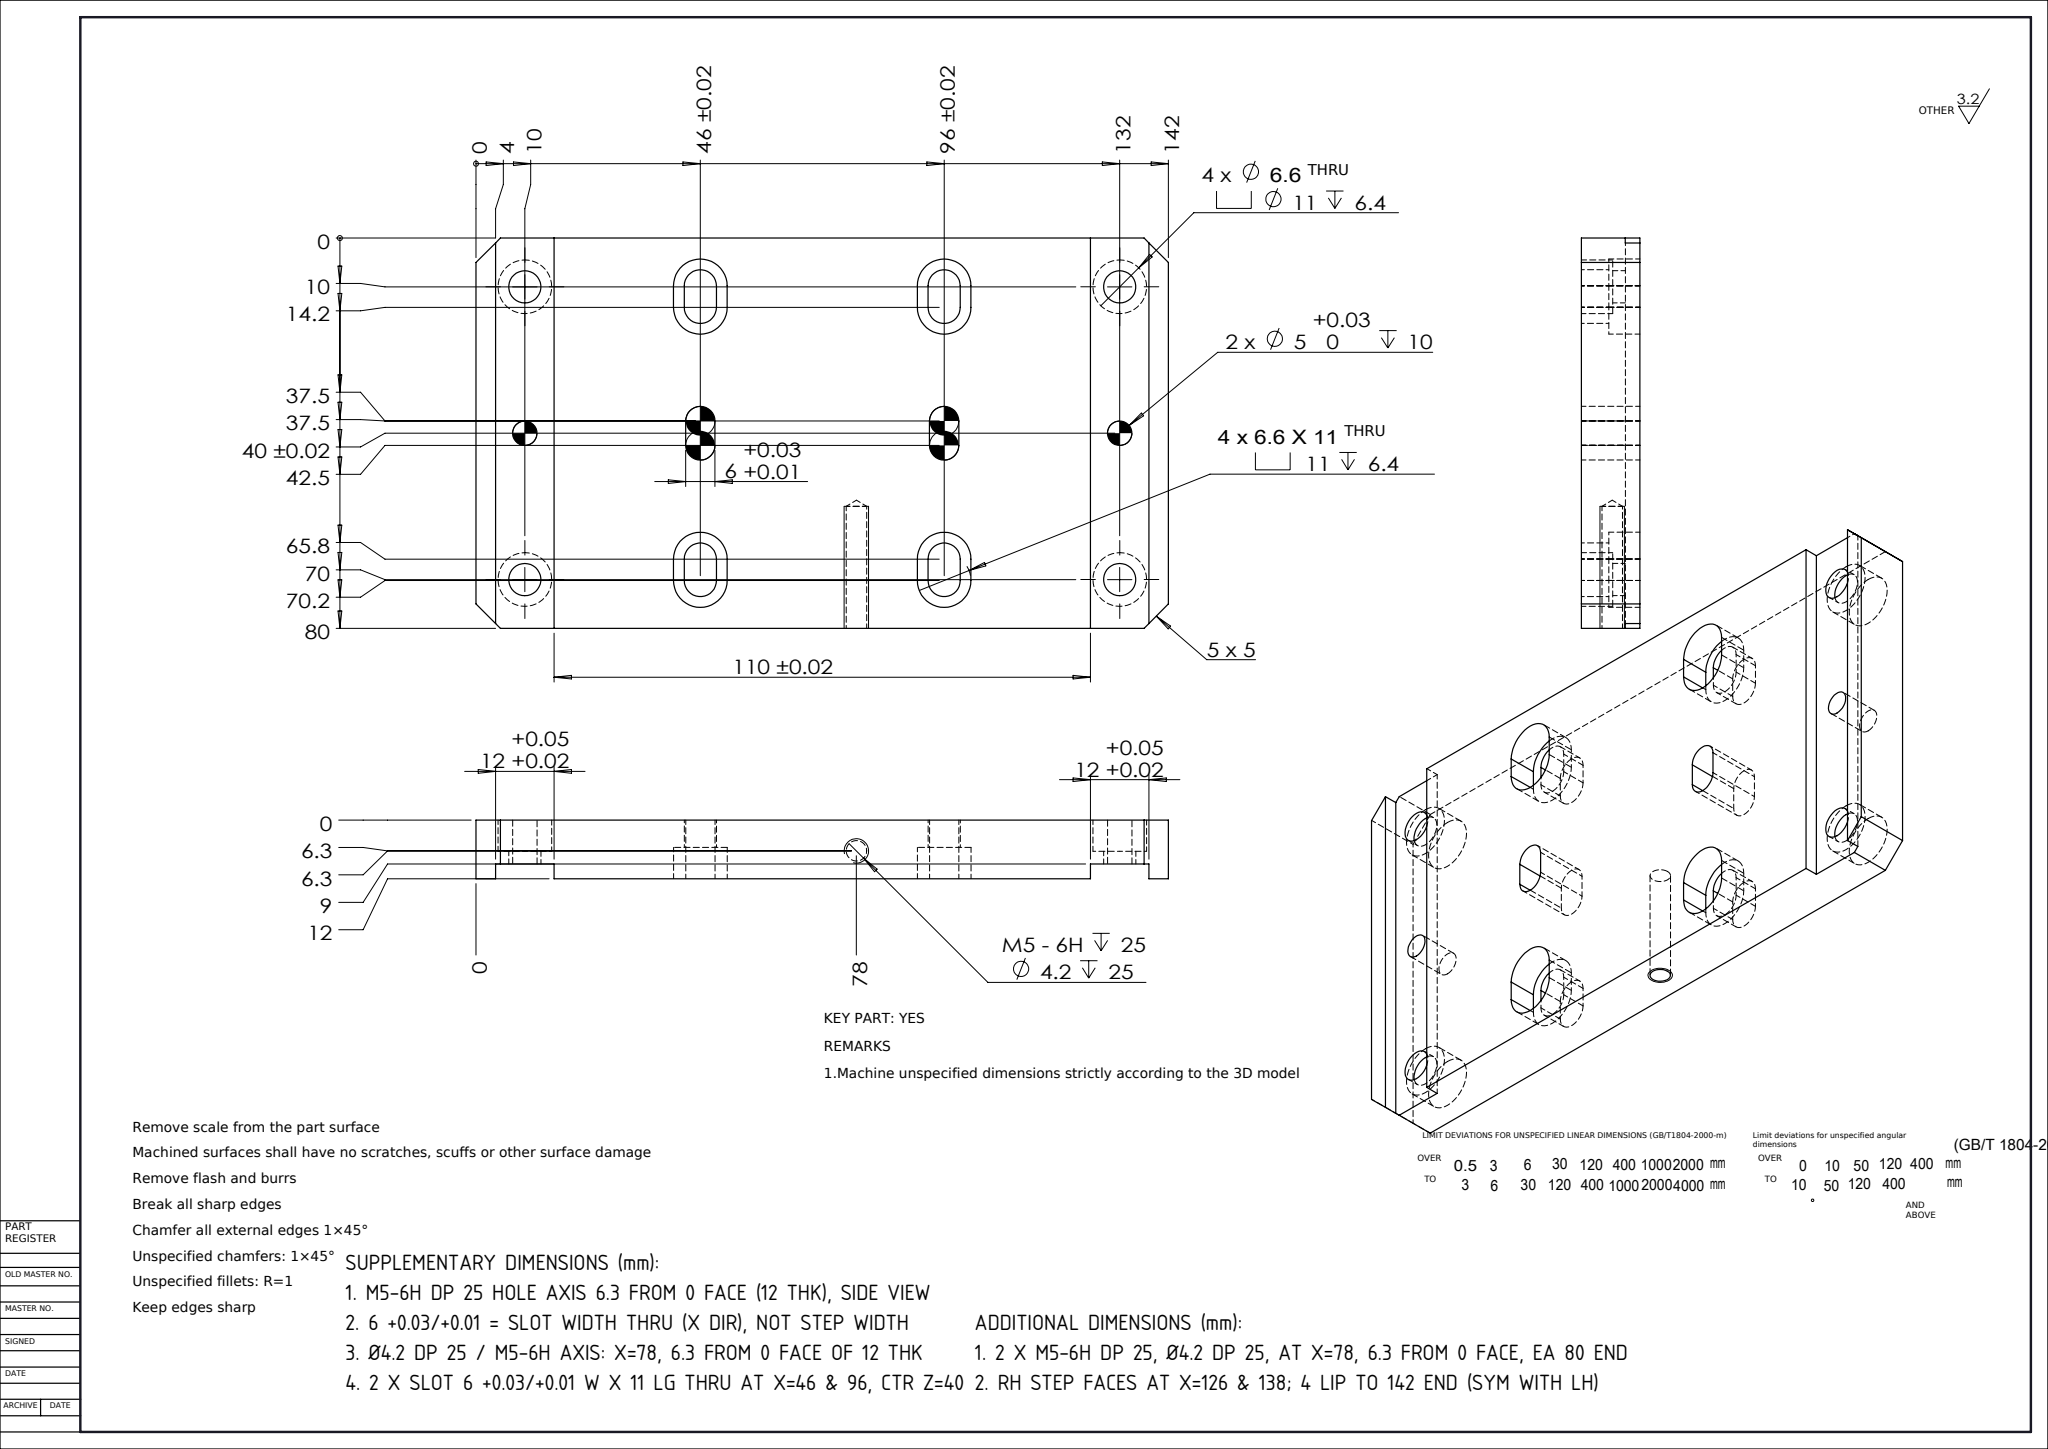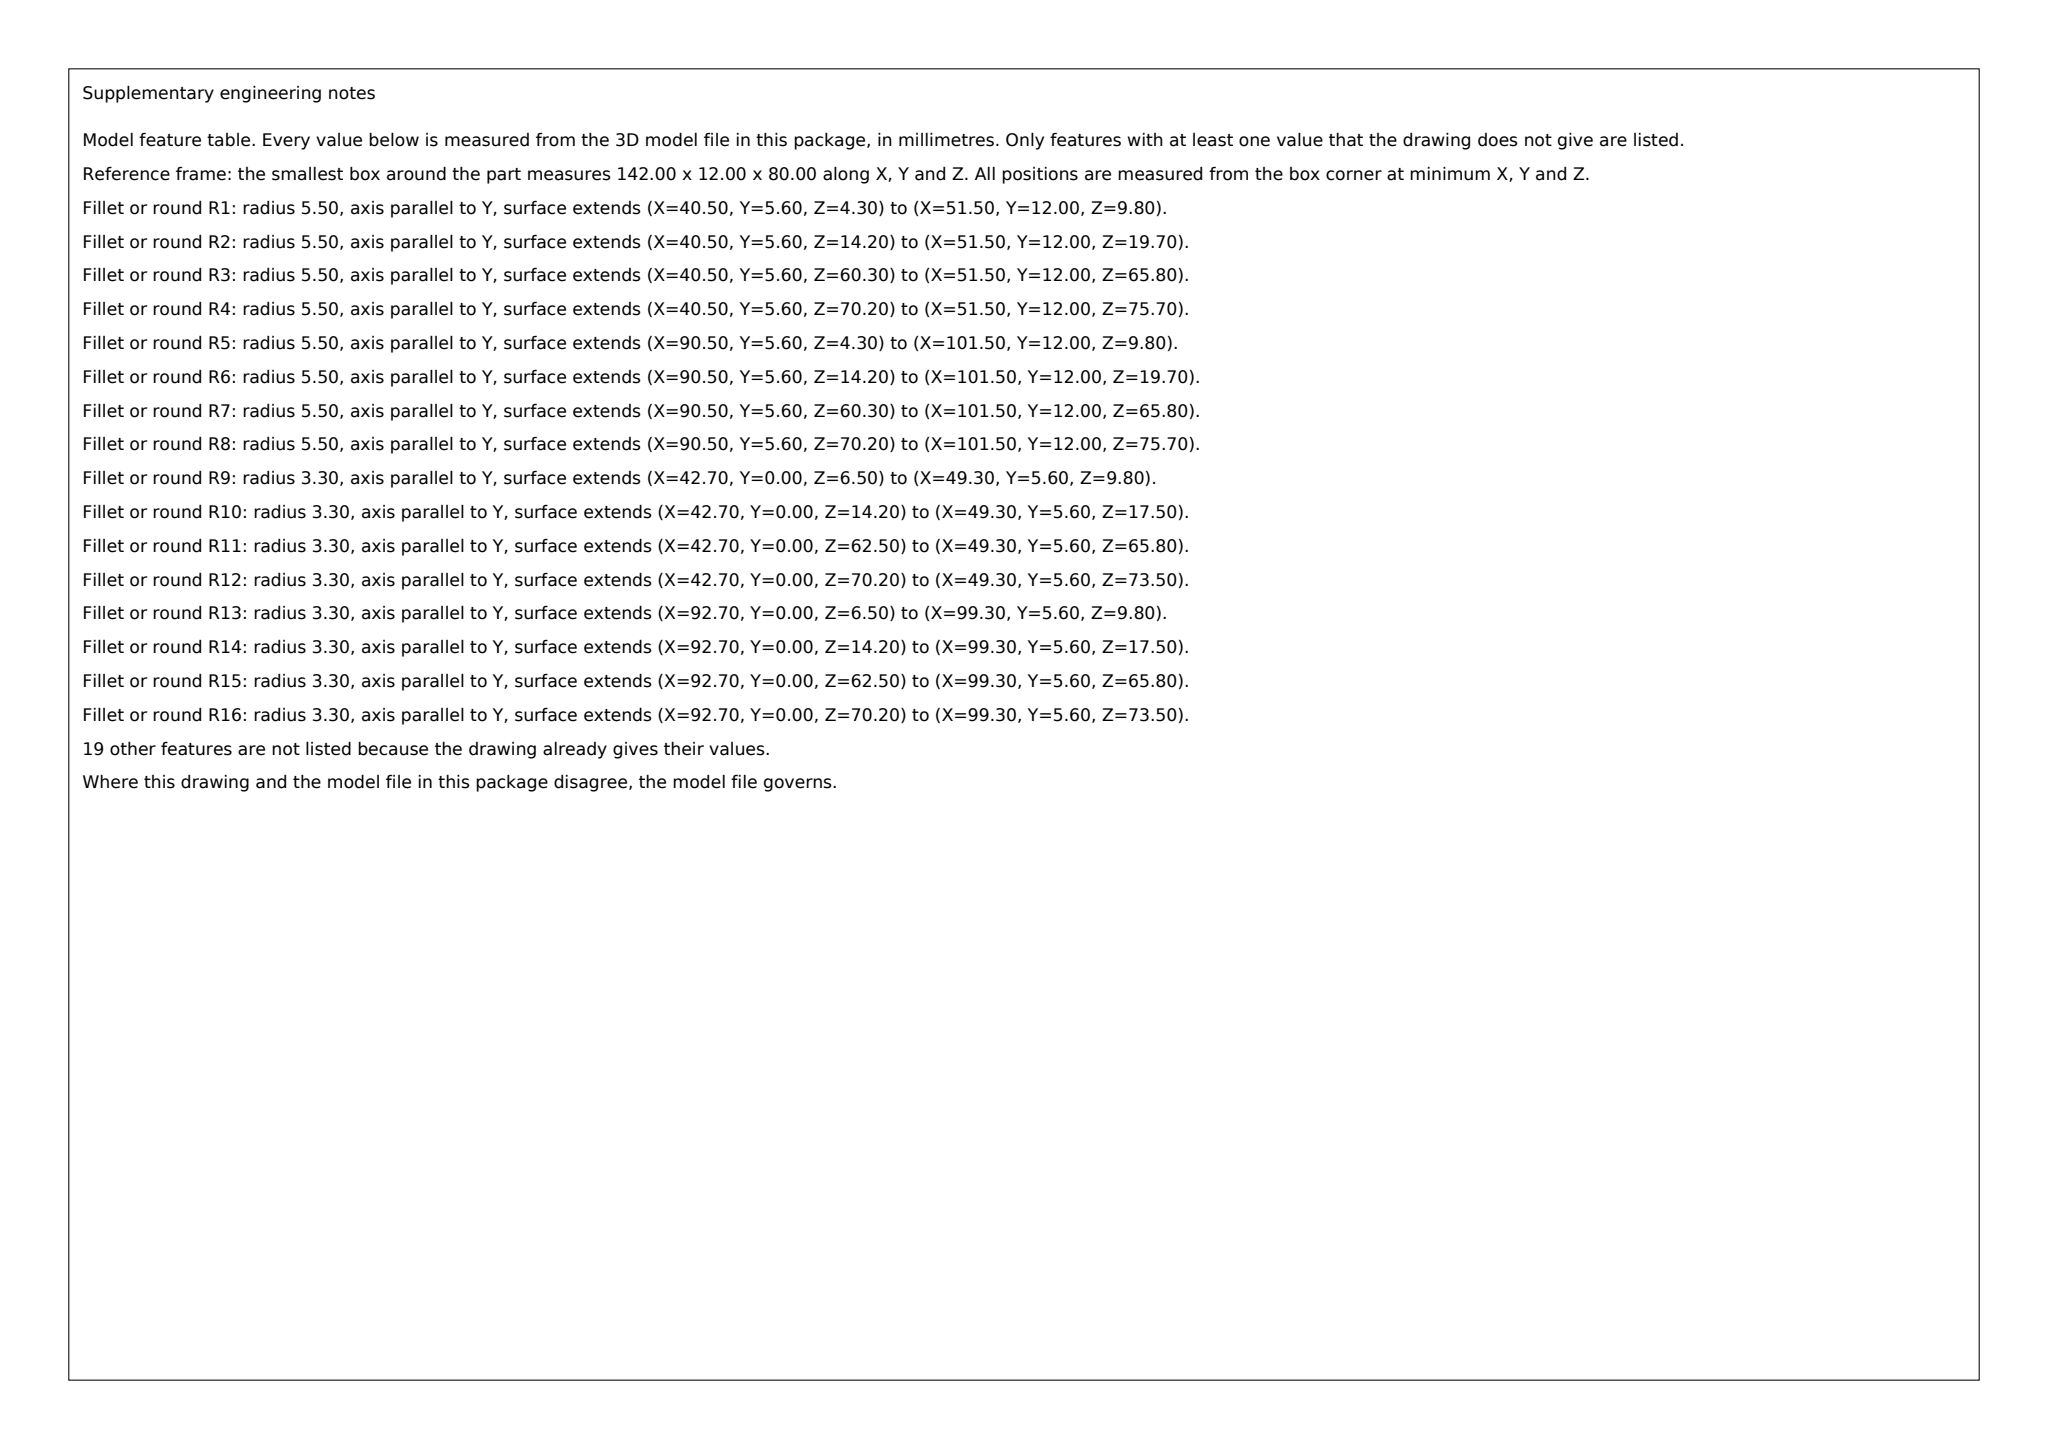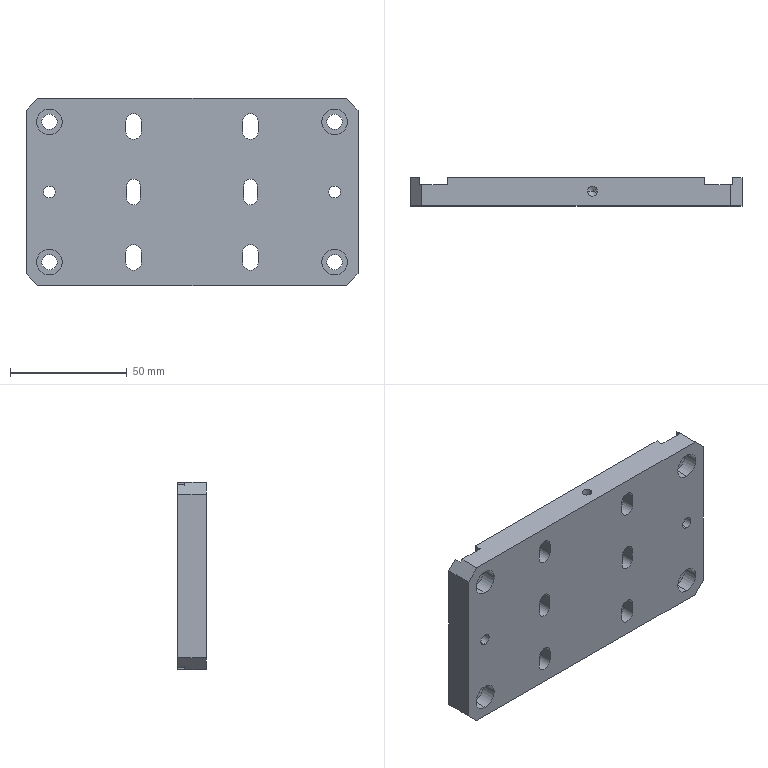Part | SolidWorks | mm | 1 solid | 100 faces | box 142 x 12 x 80 mm | volume 119984 mm3 | cylinder 52 | plane 46 | cone 2 | commonest cylinder face diameters 11 x20 6.6 x20 6 x6 5 x4 4.2 x2